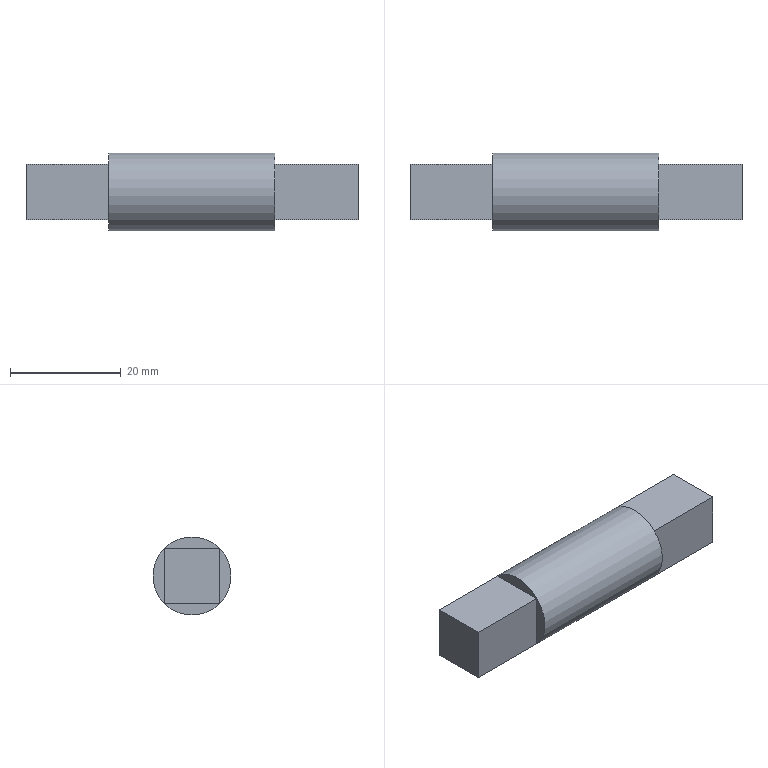Component | NX | 4 | 1 solid | 19 faces | box 60 x 14.14 x 14.14 mm | volume 7712 mm3 | plane 18 | cylinder 1 | commonest cylinder face diameters 14.142 x1
STEP:
#1=CARTESIAN_POINT('',(0.,0.,0.));
#2=DIRECTION('',(0.,0.,1.));
#3=DIRECTION('',(1.,0.,0.));
#4=AXIS2_PLACEMENT_3D('',#1,#2,#3);
#5=CARTESIAN_POINT('',(-30.,5.,43.));
#6=VERTEX_POINT('',#5);
#7=CARTESIAN_POINT('',(-15.,5.,43.));
#8=VERTEX_POINT('',#7);
#9=CARTESIAN_POINT('',(-30.,5.,43.));
#10=DIRECTION('',(1.,0.,0.));
#11=VECTOR('',#10,1.);
#12=LINE('',#9,#11);
#13=CARTESIAN_POINT('',(-30.,5.,43.));
#14=DIRECTION('',(0.,-1.,0.));
#15=DIRECTION('',(0.,0.,-1.));
#16=AXIS2_PLACEMENT_3D('',#13,#14,#15);
#17=PLANE('',#16);
#18=CARTESIAN_POINT('',(0.,0.));
#19=DIRECTION('',(0.,1.));
#20=VECTOR('',#19,1.);
#21=LINE('',#18,#20);
#22=(GEOMETRIC_REPRESENTATION_CONTEXT(2)PARAMETRIC_REPRESENTATION_CONTEXT()REPRESENTATION_CONTEXT('',''));
#23=DEFINITIONAL_REPRESENTATION('',(#21),#22);
#24=PCURVE('',#17,#23);
#25=CARTESIAN_POINT('',(-30.,-5.,43.));
#26=DIRECTION('',(0.,0.,-1.));
#27=DIRECTION('',(0.,1.,0.));
#28=AXIS2_PLACEMENT_3D('',#25,#26,#27);
#29=PLANE('',#28);
#30=CARTESIAN_POINT('',(10.,0.));
#31=DIRECTION('',(0.,1.));
#32=VECTOR('',#31,1.);
#33=LINE('',#30,#32);
#34=(GEOMETRIC_REPRESENTATION_CONTEXT(2)PARAMETRIC_REPRESENTATION_CONTEXT()REPRESENTATION_CONTEXT('',''));
#35=DEFINITIONAL_REPRESENTATION('',(#33),#34);
#36=PCURVE('',#29,#35);
#37=SURFACE_CURVE('',#12,(#24,#36),.PCURVE_S1.);
#38=EDGE_CURVE('',#6,#8,#37,.T.);
#39=ORIENTED_EDGE('',*,*,#38,.T.);
#40=CARTESIAN_POINT('',(-15.,5.,33.));
#41=VERTEX_POINT('',#40);
#42=CARTESIAN_POINT('',(-15.,5.,43.));
#43=DIRECTION('',(0.,0.,-1.));
#44=VECTOR('',#43,1.);
#45=LINE('',#42,#44);
#46=CARTESIAN_POINT('',(0.,15.));
#47=DIRECTION('',(1.,0.));
#48=VECTOR('',#47,1.);
#49=LINE('',#46,#48);
#50=(GEOMETRIC_REPRESENTATION_CONTEXT(2)PARAMETRIC_REPRESENTATION_CONTEXT()REPRESENTATION_CONTEXT('',''));
#51=DEFINITIONAL_REPRESENTATION('',(#49),#50);
#52=PCURVE('',#17,#51);
#53=CARTESIAN_POINT('',(-15.,0.,38.));
#54=DIRECTION('',(-1.,0.,0.));
#55=DIRECTION('',(0.,0.,-1.));
#56=AXIS2_PLACEMENT_3D('',#53,#54,#55);
#57=PLANE('',#56);
#58=CARTESIAN_POINT('',(-5.,-5.));
#59=DIRECTION('',(1.,0.));
#60=VECTOR('',#59,1.);
#61=LINE('',#58,#60);
#62=(GEOMETRIC_REPRESENTATION_CONTEXT(2)PARAMETRIC_REPRESENTATION_CONTEXT()REPRESENTATION_CONTEXT('',''));
#63=DEFINITIONAL_REPRESENTATION('',(#61),#62);
#64=PCURVE('',#57,#63);
#65=SURFACE_CURVE('',#45,(#52,#64),.PCURVE_S1.);
#66=EDGE_CURVE('',#8,#41,#65,.T.);
#67=ORIENTED_EDGE('',*,*,#66,.T.);
#68=CARTESIAN_POINT('',(-30.,5.,33.));
#69=VERTEX_POINT('',#68);
#70=CARTESIAN_POINT('',(-30.,5.,33.));
#71=DIRECTION('',(1.,0.,0.));
#72=VECTOR('',#71,1.);
#73=LINE('',#70,#72);
#74=CARTESIAN_POINT('',(10.,0.));
#75=DIRECTION('',(0.,1.));
#76=VECTOR('',#75,1.);
#77=LINE('',#74,#76);
#78=(GEOMETRIC_REPRESENTATION_CONTEXT(2)PARAMETRIC_REPRESENTATION_CONTEXT()REPRESENTATION_CONTEXT('',''));
#79=DEFINITIONAL_REPRESENTATION('',(#77),#78);
#80=PCURVE('',#17,#79);
#81=CARTESIAN_POINT('',(-30.,5.,33.));
#82=DIRECTION('',(0.,0.,1.));
#83=DIRECTION('',(0.,-1.,0.));
#84=AXIS2_PLACEMENT_3D('',#81,#82,#83);
#85=PLANE('',#84);
#86=CARTESIAN_POINT('',(0.,0.));
#87=DIRECTION('',(0.,1.));
#88=VECTOR('',#87,1.);
#89=LINE('',#86,#88);
#90=(GEOMETRIC_REPRESENTATION_CONTEXT(2)PARAMETRIC_REPRESENTATION_CONTEXT()REPRESENTATION_CONTEXT('',''));
#91=DEFINITIONAL_REPRESENTATION('',(#89),#90);
#92=PCURVE('',#85,#91);
#93=SURFACE_CURVE('',#73,(#80,#92),.PCURVE_S1.);
#94=EDGE_CURVE('',#69,#41,#93,.T.);
#95=ORIENTED_EDGE('',*,*,#94,.F.);
#96=CARTESIAN_POINT('',(-30.,5.,43.));
#97=DIRECTION('',(0.,0.,-1.));
#98=VECTOR('',#97,1.);
#99=LINE('',#96,#98);
#100=CARTESIAN_POINT('',(0.,0.));
#101=DIRECTION('',(1.,0.));
#102=VECTOR('',#101,1.);
#103=LINE('',#100,#102);
#104=(GEOMETRIC_REPRESENTATION_CONTEXT(2)PARAMETRIC_REPRESENTATION_CONTEXT()REPRESENTATION_CONTEXT('',''));
#105=DEFINITIONAL_REPRESENTATION('',(#103),#104);
#106=PCURVE('',#17,#105);
#107=CARTESIAN_POINT('',(-30.,0.,38.));
#108=DIRECTION('',(-1.,0.,0.));
#109=DIRECTION('',(0.,0.,-1.));
#110=AXIS2_PLACEMENT_3D('',#107,#108,#109);
#111=PLANE('',#110);
#112=CARTESIAN_POINT('',(-5.,-5.));
#113=DIRECTION('',(1.,0.));
#114=VECTOR('',#113,1.);
#115=LINE('',#112,#114);
#116=(GEOMETRIC_REPRESENTATION_CONTEXT(2)PARAMETRIC_REPRESENTATION_CONTEXT()REPRESENTATION_CONTEXT('',''));
#117=DEFINITIONAL_REPRESENTATION('',(#115),#116);
#118=PCURVE('',#111,#117);
#119=SURFACE_CURVE('',#99,(#106,#118),.PCURVE_S1.);
#120=EDGE_CURVE('',#6,#69,#119,.T.);
#121=ORIENTED_EDGE('',*,*,#120,.F.);
#122=EDGE_LOOP('',(#39,#67,#95,#121));
#123=FACE_BOUND('',#122,.T.);
#124=ADVANCED_FACE('',(#123),#17,.F.);
#125=ORIENTED_EDGE('',*,*,#94,.T.);
#126=CARTESIAN_POINT('',(-15.,-5.,33.));
#127=VERTEX_POINT('',#126);
#128=CARTESIAN_POINT('',(-15.,5.,33.));
#129=DIRECTION('',(0.,-1.,0.));
#130=VECTOR('',#129,1.);
#131=LINE('',#128,#130);
#132=CARTESIAN_POINT('',(0.,15.));
#133=DIRECTION('',(1.,0.));
#134=VECTOR('',#133,1.);
#135=LINE('',#132,#134);
#136=(GEOMETRIC_REPRESENTATION_CONTEXT(2)PARAMETRIC_REPRESENTATION_CONTEXT()REPRESENTATION_CONTEXT('',''));
#137=DEFINITIONAL_REPRESENTATION('',(#135),#136);
#138=PCURVE('',#85,#137);
#139=CARTESIAN_POINT('',(-15.,0.,38.));
#140=DIRECTION('',(-1.,0.,0.));
#141=DIRECTION('',(0.,0.,-1.));
#142=AXIS2_PLACEMENT_3D('',#139,#140,#141);
#143=PLANE('',#142);
#144=CARTESIAN_POINT('',(5.,-5.));
#145=DIRECTION('',(0.,1.));
#146=VECTOR('',#145,1.);
#147=LINE('',#144,#146);
#148=(GEOMETRIC_REPRESENTATION_CONTEXT(2)PARAMETRIC_REPRESENTATION_CONTEXT()REPRESENTATION_CONTEXT('',''));
#149=DEFINITIONAL_REPRESENTATION('',(#147),#148);
#150=PCURVE('',#143,#149);
#151=SURFACE_CURVE('',#131,(#138,#150),.PCURVE_S1.);
#152=EDGE_CURVE('',#41,#127,#151,.T.);
#153=ORIENTED_EDGE('',*,*,#152,.T.);
#154=CARTESIAN_POINT('',(-30.,-5.,33.));
#155=VERTEX_POINT('',#154);
#156=CARTESIAN_POINT('',(-30.,-5.,33.));
#157=DIRECTION('',(1.,0.,0.));
#158=VECTOR('',#157,1.);
#159=LINE('',#156,#158);
#160=CARTESIAN_POINT('',(10.,0.));
#161=DIRECTION('',(0.,1.));
#162=VECTOR('',#161,1.);
#163=LINE('',#160,#162);
#164=(GEOMETRIC_REPRESENTATION_CONTEXT(2)PARAMETRIC_REPRESENTATION_CONTEXT()REPRESENTATION_CONTEXT('',''));
#165=DEFINITIONAL_REPRESENTATION('',(#163),#164);
#166=PCURVE('',#85,#165);
#167=CARTESIAN_POINT('',(-30.,-5.,33.));
#168=DIRECTION('',(0.,1.,0.));
#169=DIRECTION('',(0.,0.,1.));
#170=AXIS2_PLACEMENT_3D('',#167,#168,#169);
#171=PLANE('',#170);
#172=CARTESIAN_POINT('',(0.,0.));
#173=DIRECTION('',(0.,1.));
#174=VECTOR('',#173,1.);
#175=LINE('',#172,#174);
#176=(GEOMETRIC_REPRESENTATION_CONTEXT(2)PARAMETRIC_REPRESENTATION_CONTEXT()REPRESENTATION_CONTEXT('',''));
#177=DEFINITIONAL_REPRESENTATION('',(#175),#176);
#178=PCURVE('',#171,#177);
#179=SURFACE_CURVE('',#159,(#166,#178),.PCURVE_S1.);
#180=EDGE_CURVE('',#155,#127,#179,.T.);
#181=ORIENTED_EDGE('',*,*,#180,.F.);
#182=CARTESIAN_POINT('',(-30.,5.,33.));
#183=DIRECTION('',(0.,-1.,0.));
#184=VECTOR('',#183,1.);
#185=LINE('',#182,#184);
#186=CARTESIAN_POINT('',(0.,0.));
#187=DIRECTION('',(1.,0.));
#188=VECTOR('',#187,1.);
#189=LINE('',#186,#188);
#190=(GEOMETRIC_REPRESENTATION_CONTEXT(2)PARAMETRIC_REPRESENTATION_CONTEXT()REPRESENTATION_CONTEXT('',''));
#191=DEFINITIONAL_REPRESENTATION('',(#189),#190);
#192=PCURVE('',#85,#191);
#193=CARTESIAN_POINT('',(5.,-5.));
#194=DIRECTION('',(0.,1.));
#195=VECTOR('',#194,1.);
#196=LINE('',#193,#195);
#197=(GEOMETRIC_REPRESENTATION_CONTEXT(2)PARAMETRIC_REPRESENTATION_CONTEXT()REPRESENTATION_CONTEXT('',''));
#198=DEFINITIONAL_REPRESENTATION('',(#196),#197);
#199=PCURVE('',#111,#198);
#200=SURFACE_CURVE('',#185,(#192,#199),.PCURVE_S1.);
#201=EDGE_CURVE('',#69,#155,#200,.T.);
#202=ORIENTED_EDGE('',*,*,#201,.F.);
#203=EDGE_LOOP('',(#125,#153,#181,#202));
#204=FACE_BOUND('',#203,.T.);
#205=ADVANCED_FACE('',(#204),#85,.F.);
#206=ORIENTED_EDGE('',*,*,#180,.T.);
#207=CARTESIAN_POINT('',(-15.,-5.,43.));
#208=VERTEX_POINT('',#207);
#209=CARTESIAN_POINT('',(-15.,-5.,33.));
#210=DIRECTION('',(0.,0.,1.));
#211=VECTOR('',#210,1.);
#212=LINE('',#209,#211);
#213=CARTESIAN_POINT('',(0.,15.));
#214=DIRECTION('',(1.,0.));
#215=VECTOR('',#214,1.);
#216=LINE('',#213,#215);
#217=(GEOMETRIC_REPRESENTATION_CONTEXT(2)PARAMETRIC_REPRESENTATION_CONTEXT()REPRESENTATION_CONTEXT('',''));
#218=DEFINITIONAL_REPRESENTATION('',(#216),#217);
#219=PCURVE('',#171,#218);
#220=CARTESIAN_POINT('',(-15.,0.,38.));
#221=DIRECTION('',(-1.,0.,0.));
#222=DIRECTION('',(0.,0.,-1.));
#223=AXIS2_PLACEMENT_3D('',#220,#221,#222);
#224=PLANE('',#223);
#225=CARTESIAN_POINT('',(5.,5.));
#226=DIRECTION('',(-1.,0.));
#227=VECTOR('',#226,1.);
#228=LINE('',#225,#227);
#229=(GEOMETRIC_REPRESENTATION_CONTEXT(2)PARAMETRIC_REPRESENTATION_CONTEXT()REPRESENTATION_CONTEXT('',''));
#230=DEFINITIONAL_REPRESENTATION('',(#228),#229);
#231=PCURVE('',#224,#230);
#232=SURFACE_CURVE('',#212,(#219,#231),.PCURVE_S1.);
#233=EDGE_CURVE('',#127,#208,#232,.T.);
#234=ORIENTED_EDGE('',*,*,#233,.T.);
#235=CARTESIAN_POINT('',(-30.,-5.,43.));
#236=VERTEX_POINT('',#235);
#237=CARTESIAN_POINT('',(-30.,-5.,43.));
#238=DIRECTION('',(1.,0.,0.));
#239=VECTOR('',#238,1.);
#240=LINE('',#237,#239);
#241=CARTESIAN_POINT('',(10.,0.));
#242=DIRECTION('',(0.,1.));
#243=VECTOR('',#242,1.);
#244=LINE('',#241,#243);
#245=(GEOMETRIC_REPRESENTATION_CONTEXT(2)PARAMETRIC_REPRESENTATION_CONTEXT()REPRESENTATION_CONTEXT('',''));
#246=DEFINITIONAL_REPRESENTATION('',(#244),#245);
#247=PCURVE('',#171,#246);
#248=CARTESIAN_POINT('',(0.,0.));
#249=DIRECTION('',(0.,1.));
#250=VECTOR('',#249,1.);
#251=LINE('',#248,#250);
#252=(GEOMETRIC_REPRESENTATION_CONTEXT(2)PARAMETRIC_REPRESENTATION_CONTEXT()REPRESENTATION_CONTEXT('',''));
#253=DEFINITIONAL_REPRESENTATION('',(#251),#252);
#254=PCURVE('',#29,#253);
#255=SURFACE_CURVE('',#240,(#247,#254),.PCURVE_S1.);
#256=EDGE_CURVE('',#236,#208,#255,.T.);
#257=ORIENTED_EDGE('',*,*,#256,.F.);
#258=CARTESIAN_POINT('',(-30.,-5.,33.));
#259=DIRECTION('',(0.,0.,1.));
#260=VECTOR('',#259,1.);
#261=LINE('',#258,#260);
#262=CARTESIAN_POINT('',(0.,0.));
#263=DIRECTION('',(1.,0.));
#264=VECTOR('',#263,1.);
#265=LINE('',#262,#264);
#266=(GEOMETRIC_REPRESENTATION_CONTEXT(2)PARAMETRIC_REPRESENTATION_CONTEXT()REPRESENTATION_CONTEXT('',''));
#267=DEFINITIONAL_REPRESENTATION('',(#265),#266);
#268=PCURVE('',#171,#267);
#269=CARTESIAN_POINT('',(5.,5.));
#270=DIRECTION('',(-1.,0.));
#271=VECTOR('',#270,1.);
#272=LINE('',#269,#271);
#273=(GEOMETRIC_REPRESENTATION_CONTEXT(2)PARAMETRIC_REPRESENTATION_CONTEXT()REPRESENTATION_CONTEXT('',''));
#274=DEFINITIONAL_REPRESENTATION('',(#272),#273);
#275=PCURVE('',#111,#274);
#276=SURFACE_CURVE('',#261,(#268,#275),.PCURVE_S1.);
#277=EDGE_CURVE('',#155,#236,#276,.T.);
#278=ORIENTED_EDGE('',*,*,#277,.F.);
#279=EDGE_LOOP('',(#206,#234,#257,#278));
#280=FACE_BOUND('',#279,.T.);
#281=ADVANCED_FACE('',(#280),#171,.F.);
#282=ORIENTED_EDGE('',*,*,#256,.T.);
#283=CARTESIAN_POINT('',(-15.,-5.,43.));
#284=DIRECTION('',(0.,1.,0.));
#285=VECTOR('',#284,1.);
#286=LINE('',#283,#285);
#287=CARTESIAN_POINT('',(0.,15.));
#288=DIRECTION('',(1.,0.));
#289=VECTOR('',#288,1.);
#290=LINE('',#287,#289);
#291=(GEOMETRIC_REPRESENTATION_CONTEXT(2)PARAMETRIC_REPRESENTATION_CONTEXT()REPRESENTATION_CONTEXT('',''));
#292=DEFINITIONAL_REPRESENTATION('',(#290),#291);
#293=PCURVE('',#29,#292);
#294=CARTESIAN_POINT('',(-15.,0.,38.));
#295=DIRECTION('',(-1.,0.,0.));
#296=DIRECTION('',(0.,0.,-1.));
#297=AXIS2_PLACEMENT_3D('',#294,#295,#296);
#298=PLANE('',#297);
#299=CARTESIAN_POINT('',(-5.,5.));
#300=DIRECTION('',(0.,-1.));
#301=VECTOR('',#300,1.);
#302=LINE('',#299,#301);
#303=(GEOMETRIC_REPRESENTATION_CONTEXT(2)PARAMETRIC_REPRESENTATION_CONTEXT()REPRESENTATION_CONTEXT('',''));
#304=DEFINITIONAL_REPRESENTATION('',(#302),#303);
#305=PCURVE('',#298,#304);
#306=SURFACE_CURVE('',#286,(#293,#305),.PCURVE_S1.);
#307=EDGE_CURVE('',#208,#8,#306,.T.);
#308=ORIENTED_EDGE('',*,*,#307,.T.);
#309=ORIENTED_EDGE('',*,*,#38,.F.);
#310=CARTESIAN_POINT('',(-30.,-5.,43.));
#311=DIRECTION('',(0.,1.,0.));
#312=VECTOR('',#311,1.);
#313=LINE('',#310,#312);
#314=CARTESIAN_POINT('',(0.,0.));
#315=DIRECTION('',(1.,0.));
#316=VECTOR('',#315,1.);
#317=LINE('',#314,#316);
#318=(GEOMETRIC_REPRESENTATION_CONTEXT(2)PARAMETRIC_REPRESENTATION_CONTEXT()REPRESENTATION_CONTEXT('',''));
#319=DEFINITIONAL_REPRESENTATION('',(#317),#318);
#320=PCURVE('',#29,#319);
#321=CARTESIAN_POINT('',(-5.,5.));
#322=DIRECTION('',(0.,-1.));
#323=VECTOR('',#322,1.);
#324=LINE('',#321,#323);
#325=(GEOMETRIC_REPRESENTATION_CONTEXT(2)PARAMETRIC_REPRESENTATION_CONTEXT()REPRESENTATION_CONTEXT('',''));
#326=DEFINITIONAL_REPRESENTATION('',(#324),#325);
#327=PCURVE('',#111,#326);
#328=SURFACE_CURVE('',#313,(#320,#327),.PCURVE_S1.);
#329=EDGE_CURVE('',#236,#6,#328,.T.);
#330=ORIENTED_EDGE('',*,*,#329,.F.);
#331=EDGE_LOOP('',(#282,#308,#309,#330));
#332=FACE_BOUND('',#331,.T.);
#333=ADVANCED_FACE('',(#332),#29,.F.);
#334=ORIENTED_EDGE('',*,*,#120,.T.);
#335=ORIENTED_EDGE('',*,*,#201,.T.);
#336=ORIENTED_EDGE('',*,*,#277,.T.);
#337=ORIENTED_EDGE('',*,*,#329,.T.);
#338=EDGE_LOOP('',(#334,#335,#336,#337));
#339=FACE_BOUND('',#338,.T.);
#340=ADVANCED_FACE('',(#339),#111,.T.);
#341=ORIENTED_EDGE('',*,*,#66,.F.);
#342=CARTESIAN_POINT('',(-15.,0.,38.));
#343=DIRECTION('',(1.,0.,0.));
#344=DIRECTION('',(0.,0.,-1.));
#345=AXIS2_PLACEMENT_3D('',#342,#343,#344);
#346=CIRCLE('',#345,7.071);
#347=CARTESIAN_POINT('',(7.071,0.));
#348=CARTESIAN_POINT('',(7.071,-12.247));
#349=CARTESIAN_POINT('',(-3.536,-6.124));
#350=CARTESIAN_POINT('',(-14.142,-0.));
#351=CARTESIAN_POINT('',(-3.536,6.124));
#352=CARTESIAN_POINT('',(7.071,12.247));
#353=CARTESIAN_POINT('',(7.071,0.));
#354=(BOUNDED_CURVE()B_SPLINE_CURVE(2,(#347,#348,#349,#350,#351,#352,#353),.UNSPECIFIED.,.T.,.F.)B_SPLINE_CURVE_WITH_KNOTS((1,2,2,2,2,1),(-2.094,0.,2.094,4.189,6.283,8.378),.UNSPECIFIED.)CURVE()GEOMETRIC_REPRESENTATION_ITEM()RATIONAL_B_SPLINE_CURVE((1.,0.5,1.,0.5,1.,0.5,1.))REPRESENTATION_ITEM(''));
#355=(GEOMETRIC_REPRESENTATION_CONTEXT(2)PARAMETRIC_REPRESENTATION_CONTEXT()REPRESENTATION_CONTEXT('',''));
#356=DEFINITIONAL_REPRESENTATION('',(#354),#355);
#357=PCURVE('',#57,#356);
#358=CARTESIAN_POINT('',(30.,0.,38.));
#359=DIRECTION('',(-1.,0.,0.));
#360=DIRECTION('',(0.,0.,1.));
#361=AXIS2_PLACEMENT_3D('',#358,#359,#360);
#362=CYLINDRICAL_SURFACE('',#361,7.071);
#363=CARTESIAN_POINT('',(3.142,45.));
#364=DIRECTION('',(-1.,0.));
#365=VECTOR('',#364,1.);
#366=LINE('',#363,#365);
#367=(GEOMETRIC_REPRESENTATION_CONTEXT(2)PARAMETRIC_REPRESENTATION_CONTEXT()REPRESENTATION_CONTEXT('',''));
#368=DEFINITIONAL_REPRESENTATION('',(#366),#367);
#369=PCURVE('',#362,#368);
#370=SURFACE_CURVE('',#346,(#357,#369),.PCURVE_S1.);
#371=EDGE_CURVE('',#41,#8,#370,.T.);
#372=ORIENTED_EDGE('',*,*,#371,.F.);
#373=EDGE_LOOP('',(#341,#372));
#374=FACE_BOUND('',#373,.T.);
#375=ADVANCED_FACE('',(#374),#57,.T.);
#376=ORIENTED_EDGE('',*,*,#152,.F.);
#377=CARTESIAN_POINT('',(-15.,0.,38.));
#378=DIRECTION('',(1.,0.,0.));
#379=DIRECTION('',(0.,0.,-1.));
#380=AXIS2_PLACEMENT_3D('',#377,#378,#379);
#381=CIRCLE('',#380,7.071);
#382=CARTESIAN_POINT('',(7.071,0.));
#383=CARTESIAN_POINT('',(7.071,-12.247));
#384=CARTESIAN_POINT('',(-3.536,-6.124));
#385=CARTESIAN_POINT('',(-14.142,-0.));
#386=CARTESIAN_POINT('',(-3.536,6.124));
#387=CARTESIAN_POINT('',(7.071,12.247));
#388=CARTESIAN_POINT('',(7.071,0.));
#389=(BOUNDED_CURVE()B_SPLINE_CURVE(2,(#382,#383,#384,#385,#386,#387,#388),.UNSPECIFIED.,.T.,.F.)B_SPLINE_CURVE_WITH_KNOTS((1,2,2,2,2,1),(-2.094,0.,2.094,4.189,6.283,8.378),.UNSPECIFIED.)CURVE()GEOMETRIC_REPRESENTATION_ITEM()RATIONAL_B_SPLINE_CURVE((1.,0.5,1.,0.5,1.,0.5,1.))REPRESENTATION_ITEM(''));
#390=(GEOMETRIC_REPRESENTATION_CONTEXT(2)PARAMETRIC_REPRESENTATION_CONTEXT()REPRESENTATION_CONTEXT('',''));
#391=DEFINITIONAL_REPRESENTATION('',(#389),#390);
#392=PCURVE('',#143,#391);
#393=CARTESIAN_POINT('',(9.425,45.));
#394=DIRECTION('',(-1.,0.));
#395=VECTOR('',#394,1.);
#396=LINE('',#393,#395);
#397=(GEOMETRIC_REPRESENTATION_CONTEXT(2)PARAMETRIC_REPRESENTATION_CONTEXT()REPRESENTATION_CONTEXT('',''));
#398=DEFINITIONAL_REPRESENTATION('',(#396),#397);
#399=PCURVE('',#362,#398);
#400=SURFACE_CURVE('',#381,(#392,#399),.PCURVE_S1.);
#401=EDGE_CURVE('',#127,#41,#400,.T.);
#402=ORIENTED_EDGE('',*,*,#401,.F.);
#403=EDGE_LOOP('',(#376,#402));
#404=FACE_BOUND('',#403,.T.);
#405=ADVANCED_FACE('',(#404),#143,.T.);
#406=ORIENTED_EDGE('',*,*,#233,.F.);
#407=CARTESIAN_POINT('',(-15.,0.,38.));
#408=DIRECTION('',(1.,0.,0.));
#409=DIRECTION('',(0.,0.,-1.));
#410=AXIS2_PLACEMENT_3D('',#407,#408,#409);
#411=CIRCLE('',#410,7.071);
#412=CARTESIAN_POINT('',(7.071,0.));
#413=CARTESIAN_POINT('',(7.071,-12.247));
#414=CARTESIAN_POINT('',(-3.536,-6.124));
#415=CARTESIAN_POINT('',(-14.142,-0.));
#416=CARTESIAN_POINT('',(-3.536,6.124));
#417=CARTESIAN_POINT('',(7.071,12.247));
#418=CARTESIAN_POINT('',(7.071,0.));
#419=(BOUNDED_CURVE()B_SPLINE_CURVE(2,(#412,#413,#414,#415,#416,#417,#418),.UNSPECIFIED.,.T.,.F.)B_SPLINE_CURVE_WITH_KNOTS((1,2,2,2,2,1),(-2.094,0.,2.094,4.189,6.283,8.378),.UNSPECIFIED.)CURVE()GEOMETRIC_REPRESENTATION_ITEM()RATIONAL_B_SPLINE_CURVE((1.,0.5,1.,0.5,1.,0.5,1.))REPRESENTATION_ITEM(''));
#420=(GEOMETRIC_REPRESENTATION_CONTEXT(2)PARAMETRIC_REPRESENTATION_CONTEXT()REPRESENTATION_CONTEXT('',''));
#421=DEFINITIONAL_REPRESENTATION('',(#419),#420);
#422=PCURVE('',#224,#421);
#423=CARTESIAN_POINT('',(9.425,45.));
#424=DIRECTION('',(-1.,0.));
#425=VECTOR('',#424,1.);
#426=LINE('',#423,#425);
#427=(GEOMETRIC_REPRESENTATION_CONTEXT(2)PARAMETRIC_REPRESENTATION_CONTEXT()REPRESENTATION_CONTEXT('',''));
#428=DEFINITIONAL_REPRESENTATION('',(#426),#427);
#429=PCURVE('',#362,#428);
#430=SURFACE_CURVE('',#411,(#422,#429),.PCURVE_S1.);
#431=EDGE_CURVE('',#208,#127,#430,.T.);
#432=ORIENTED_EDGE('',*,*,#431,.F.);
#433=EDGE_LOOP('',(#406,#432));
#434=FACE_BOUND('',#433,.T.);
#435=ADVANCED_FACE('',(#434),#224,.T.);
#436=ORIENTED_EDGE('',*,*,#307,.F.);
#437=CARTESIAN_POINT('',(-15.,0.,38.));
#438=DIRECTION('',(1.,0.,0.));
#439=DIRECTION('',(0.,0.,-1.));
#440=AXIS2_PLACEMENT_3D('',#437,#438,#439);
#441=CIRCLE('',#440,7.071);
#442=CARTESIAN_POINT('',(7.071,0.));
#443=CARTESIAN_POINT('',(7.071,-12.247));
#444=CARTESIAN_POINT('',(-3.536,-6.124));
#445=CARTESIAN_POINT('',(-14.142,-0.));
#446=CARTESIAN_POINT('',(-3.536,6.124));
#447=CARTESIAN_POINT('',(7.071,12.247));
#448=CARTESIAN_POINT('',(7.071,0.));
#449=(BOUNDED_CURVE()B_SPLINE_CURVE(2,(#442,#443,#444,#445,#446,#447,#448),.UNSPECIFIED.,.T.,.F.)B_SPLINE_CURVE_WITH_KNOTS((1,2,2,2,2,1),(-2.094,0.,2.094,4.189,6.283,8.378),.UNSPECIFIED.)CURVE()GEOMETRIC_REPRESENTATION_ITEM()RATIONAL_B_SPLINE_CURVE((1.,0.5,1.,0.5,1.,0.5,1.))REPRESENTATION_ITEM(''));
#450=(GEOMETRIC_REPRESENTATION_CONTEXT(2)PARAMETRIC_REPRESENTATION_CONTEXT()REPRESENTATION_CONTEXT('',''));
#451=DEFINITIONAL_REPRESENTATION('',(#449),#450);
#452=PCURVE('',#298,#451);
#453=CARTESIAN_POINT('',(9.425,45.));
#454=DIRECTION('',(-1.,0.));
#455=VECTOR('',#454,1.);
#456=LINE('',#453,#455);
#457=(GEOMETRIC_REPRESENTATION_CONTEXT(2)PARAMETRIC_REPRESENTATION_CONTEXT()REPRESENTATION_CONTEXT('',''));
#458=DEFINITIONAL_REPRESENTATION('',(#456),#457);
#459=PCURVE('',#362,#458);
#460=SURFACE_CURVE('',#441,(#452,#459),.PCURVE_S1.);
#461=EDGE_CURVE('',#8,#208,#460,.T.);
#462=ORIENTED_EDGE('',*,*,#461,.F.);
#463=EDGE_LOOP('',(#436,#462));
#464=FACE_BOUND('',#463,.T.);
#465=ADVANCED_FACE('',(#464),#298,.T.);
#466=CARTESIAN_POINT('',(15.,5.,33.));
#467=VERTEX_POINT('',#466);
#468=CARTESIAN_POINT('',(15.,5.,43.));
#469=VERTEX_POINT('',#468);
#470=CARTESIAN_POINT('',(15.,5.,43.));
#471=DIRECTION('',(0.,0.,1.));
#472=VECTOR('',#471,1.);
#473=LINE('',#470,#472);
#474=CARTESIAN_POINT('',(15.,0.,38.));
#475=DIRECTION('',(1.,0.,0.));
#476=DIRECTION('',(0.,0.,1.));
#477=AXIS2_PLACEMENT_3D('',#474,#475,#476);
#478=PLANE('',#477);
#479=CARTESIAN_POINT('',(5.,-5.));
#480=DIRECTION('',(1.,0.));
#481=VECTOR('',#480,1.);
#482=LINE('',#479,#481);
#483=(GEOMETRIC_REPRESENTATION_CONTEXT(2)PARAMETRIC_REPRESENTATION_CONTEXT()REPRESENTATION_CONTEXT('',''));
#484=DEFINITIONAL_REPRESENTATION('',(#482),#483);
#485=PCURVE('',#478,#484);
#486=CARTESIAN_POINT('',(-30.,5.,43.));
#487=DIRECTION('',(0.,-1.,0.));
#488=DIRECTION('',(0.,0.,-1.));
#489=AXIS2_PLACEMENT_3D('',#486,#487,#488);
#490=PLANE('',#489);
#491=CARTESIAN_POINT('',(0.,45.));
#492=DIRECTION('',(-1.,0.));
#493=VECTOR('',#492,1.);
#494=LINE('',#491,#493);
#495=(GEOMETRIC_REPRESENTATION_CONTEXT(2)PARAMETRIC_REPRESENTATION_CONTEXT()REPRESENTATION_CONTEXT('',''));
#496=DEFINITIONAL_REPRESENTATION('',(#494),#495);
#497=PCURVE('',#490,#496);
#498=SURFACE_CURVE('',#473,(#485,#497),.PCURVE_S1.);
#499=EDGE_CURVE('',#467,#469,#498,.T.);
#500=ORIENTED_EDGE('',*,*,#499,.F.);
#501=CARTESIAN_POINT('',(15.,0.,38.));
#502=DIRECTION('',(-1.,0.,0.));
#503=DIRECTION('',(0.,0.,1.));
#504=AXIS2_PLACEMENT_3D('',#501,#502,#503);
#505=CIRCLE('',#504,7.071);
#506=CARTESIAN_POINT('',(7.071,0.));
#507=CARTESIAN_POINT('',(7.071,-12.247));
#508=CARTESIAN_POINT('',(-3.536,-6.124));
#509=CARTESIAN_POINT('',(-14.142,-0.));
#510=CARTESIAN_POINT('',(-3.536,6.124));
#511=CARTESIAN_POINT('',(7.071,12.247));
#512=CARTESIAN_POINT('',(7.071,0.));
#513=(BOUNDED_CURVE()B_SPLINE_CURVE(2,(#506,#507,#508,#509,#510,#511,#512),.UNSPECIFIED.,.T.,.F.)B_SPLINE_CURVE_WITH_KNOTS((1,2,2,2,2,1),(-2.094,0.,2.094,4.189,6.283,8.378),.UNSPECIFIED.)CURVE()GEOMETRIC_REPRESENTATION_ITEM()RATIONAL_B_SPLINE_CURVE((1.,0.5,1.,0.5,1.,0.5,1.))REPRESENTATION_ITEM(''));
#514=(GEOMETRIC_REPRESENTATION_CONTEXT(2)PARAMETRIC_REPRESENTATION_CONTEXT()REPRESENTATION_CONTEXT('',''));
#515=DEFINITIONAL_REPRESENTATION('',(#513),#514);
#516=PCURVE('',#478,#515);
#517=CARTESIAN_POINT('',(0.,15.));
#518=DIRECTION('',(1.,0.));
#519=VECTOR('',#518,1.);
#520=LINE('',#517,#519);
#521=(GEOMETRIC_REPRESENTATION_CONTEXT(2)PARAMETRIC_REPRESENTATION_CONTEXT()REPRESENTATION_CONTEXT('',''));
#522=DEFINITIONAL_REPRESENTATION('',(#520),#521);
#523=PCURVE('',#362,#522);
#524=SURFACE_CURVE('',#505,(#516,#523),.PCURVE_S1.);
#525=EDGE_CURVE('',#469,#467,#524,.T.);
#526=ORIENTED_EDGE('',*,*,#525,.F.);
#527=EDGE_LOOP('',(#500,#526));
#528=FACE_BOUND('',#527,.T.);
#529=ADVANCED_FACE('',(#528),#478,.T.);
#530=CARTESIAN_POINT('',(15.,-5.,33.));
#531=VERTEX_POINT('',#530);
#532=CARTESIAN_POINT('',(15.,5.,33.));
#533=DIRECTION('',(0.,1.,0.));
#534=VECTOR('',#533,1.);
#535=LINE('',#532,#534);
#536=CARTESIAN_POINT('',(15.,0.,38.));
#537=DIRECTION('',(1.,0.,0.));
#538=DIRECTION('',(0.,0.,1.));
#539=AXIS2_PLACEMENT_3D('',#536,#537,#538);
#540=PLANE('',#539);
#541=CARTESIAN_POINT('',(-5.,-5.));
#542=DIRECTION('',(0.,-1.));
#543=VECTOR('',#542,1.);
#544=LINE('',#541,#543);
#545=(GEOMETRIC_REPRESENTATION_CONTEXT(2)PARAMETRIC_REPRESENTATION_CONTEXT()REPRESENTATION_CONTEXT('',''));
#546=DEFINITIONAL_REPRESENTATION('',(#544),#545);
#547=PCURVE('',#540,#546);
#548=CARTESIAN_POINT('',(-30.,5.,33.));
#549=DIRECTION('',(0.,0.,1.));
#550=DIRECTION('',(0.,-1.,0.));
#551=AXIS2_PLACEMENT_3D('',#548,#549,#550);
#552=PLANE('',#551);
#553=CARTESIAN_POINT('',(0.,45.));
#554=DIRECTION('',(-1.,0.));
#555=VECTOR('',#554,1.);
#556=LINE('',#553,#555);
#557=(GEOMETRIC_REPRESENTATION_CONTEXT(2)PARAMETRIC_REPRESENTATION_CONTEXT()REPRESENTATION_CONTEXT('',''));
#558=DEFINITIONAL_REPRESENTATION('',(#556),#557);
#559=PCURVE('',#552,#558);
#560=SURFACE_CURVE('',#535,(#547,#559),.PCURVE_S1.);
#561=EDGE_CURVE('',#531,#467,#560,.T.);
#562=ORIENTED_EDGE('',*,*,#561,.F.);
#563=CARTESIAN_POINT('',(15.,0.,38.));
#564=DIRECTION('',(-1.,0.,0.));
#565=DIRECTION('',(0.,0.,1.));
#566=AXIS2_PLACEMENT_3D('',#563,#564,#565);
#567=CIRCLE('',#566,7.071);
#568=CARTESIAN_POINT('',(7.071,0.));
#569=CARTESIAN_POINT('',(7.071,-12.247));
#570=CARTESIAN_POINT('',(-3.536,-6.124));
#571=CARTESIAN_POINT('',(-14.142,-0.));
#572=CARTESIAN_POINT('',(-3.536,6.124));
#573=CARTESIAN_POINT('',(7.071,12.247));
#574=CARTESIAN_POINT('',(7.071,0.));
#575=(BOUNDED_CURVE()B_SPLINE_CURVE(2,(#568,#569,#570,#571,#572,#573,#574),.UNSPECIFIED.,.T.,.F.)B_SPLINE_CURVE_WITH_KNOTS((1,2,2,2,2,1),(-2.094,0.,2.094,4.189,6.283,8.378),.UNSPECIFIED.)CURVE()GEOMETRIC_REPRESENTATION_ITEM()RATIONAL_B_SPLINE_CURVE((1.,0.5,1.,0.5,1.,0.5,1.))REPRESENTATION_ITEM(''));
#576=(GEOMETRIC_REPRESENTATION_CONTEXT(2)PARAMETRIC_REPRESENTATION_CONTEXT()REPRESENTATION_CONTEXT('',''));
#577=DEFINITIONAL_REPRESENTATION('',(#575),#576);
#578=PCURVE('',#540,#577);
#579=CARTESIAN_POINT('',(0.,15.));
#580=DIRECTION('',(1.,0.));
#581=VECTOR('',#580,1.);
#582=LINE('',#579,#581);
#583=(GEOMETRIC_REPRESENTATION_CONTEXT(2)PARAMETRIC_REPRESENTATION_CONTEXT()REPRESENTATION_CONTEXT('',''));
#584=DEFINITIONAL_REPRESENTATION('',(#582),#583);
#585=PCURVE('',#362,#584);
#586=SURFACE_CURVE('',#567,(#578,#585),.PCURVE_S1.);
#587=EDGE_CURVE('',#467,#531,#586,.T.);
#588=ORIENTED_EDGE('',*,*,#587,.F.);
#589=EDGE_LOOP('',(#562,#588));
#590=FACE_BOUND('',#589,.T.);
#591=ADVANCED_FACE('',(#590),#540,.T.);
#592=CARTESIAN_POINT('',(15.,-5.,43.));
#593=VERTEX_POINT('',#592);
#594=CARTESIAN_POINT('',(15.,-5.,33.));
#595=DIRECTION('',(0.,0.,-1.));
#596=VECTOR('',#595,1.);
#597=LINE('',#594,#596);
#598=CARTESIAN_POINT('',(15.,0.,38.));
#599=DIRECTION('',(1.,0.,0.));
#600=DIRECTION('',(0.,0.,1.));
#601=AXIS2_PLACEMENT_3D('',#598,#599,#600);
#602=PLANE('',#601);
#603=CARTESIAN_POINT('',(-5.,5.));
#604=DIRECTION('',(-1.,0.));
#605=VECTOR('',#604,1.);
#606=LINE('',#603,#605);
#607=(GEOMETRIC_REPRESENTATION_CONTEXT(2)PARAMETRIC_REPRESENTATION_CONTEXT()REPRESENTATION_CONTEXT('',''));
#608=DEFINITIONAL_REPRESENTATION('',(#606),#607);
#609=PCURVE('',#602,#608);
#610=CARTESIAN_POINT('',(-30.,-5.,33.));
#611=DIRECTION('',(0.,1.,0.));
#612=DIRECTION('',(0.,0.,1.));
#613=AXIS2_PLACEMENT_3D('',#610,#611,#612);
#614=PLANE('',#613);
#615=CARTESIAN_POINT('',(0.,45.));
#616=DIRECTION('',(-1.,0.));
#617=VECTOR('',#616,1.);
#618=LINE('',#615,#617);
#619=(GEOMETRIC_REPRESENTATION_CONTEXT(2)PARAMETRIC_REPRESENTATION_CONTEXT()REPRESENTATION_CONTEXT('',''));
#620=DEFINITIONAL_REPRESENTATION('',(#618),#619);
#621=PCURVE('',#614,#620);
#622=SURFACE_CURVE('',#597,(#609,#621),.PCURVE_S1.);
#623=EDGE_CURVE('',#593,#531,#622,.T.);
#624=ORIENTED_EDGE('',*,*,#623,.F.);
#625=CARTESIAN_POINT('',(15.,0.,38.));
#626=DIRECTION('',(-1.,0.,0.));
#627=DIRECTION('',(0.,0.,1.));
#628=AXIS2_PLACEMENT_3D('',#625,#626,#627);
#629=CIRCLE('',#628,7.071);
#630=CARTESIAN_POINT('',(7.071,0.));
#631=CARTESIAN_POINT('',(7.071,-12.247));
#632=CARTESIAN_POINT('',(-3.536,-6.124));
#633=CARTESIAN_POINT('',(-14.142,-0.));
#634=CARTESIAN_POINT('',(-3.536,6.124));
#635=CARTESIAN_POINT('',(7.071,12.247));
#636=CARTESIAN_POINT('',(7.071,0.));
#637=(BOUNDED_CURVE()B_SPLINE_CURVE(2,(#630,#631,#632,#633,#634,#635,#636),.UNSPECIFIED.,.T.,.F.)B_SPLINE_CURVE_WITH_KNOTS((1,2,2,2,2,1),(-2.094,0.,2.094,4.189,6.283,8.378),.UNSPECIFIED.)CURVE()GEOMETRIC_REPRESENTATION_ITEM()RATIONAL_B_SPLINE_CURVE((1.,0.5,1.,0.5,1.,0.5,1.))REPRESENTATION_ITEM(''));
#638=(GEOMETRIC_REPRESENTATION_CONTEXT(2)PARAMETRIC_REPRESENTATION_CONTEXT()REPRESENTATION_CONTEXT('',''));
#639=DEFINITIONAL_REPRESENTATION('',(#637),#638);
#640=PCURVE('',#602,#639);
#641=CARTESIAN_POINT('',(0.,15.));
#642=DIRECTION('',(1.,0.));
#643=VECTOR('',#642,1.);
#644=LINE('',#641,#643);
#645=(GEOMETRIC_REPRESENTATION_CONTEXT(2)PARAMETRIC_REPRESENTATION_CONTEXT()REPRESENTATION_CONTEXT('',''));
#646=DEFINITIONAL_REPRESENTATION('',(#644),#645);
#647=PCURVE('',#362,#646);
#648=SURFACE_CURVE('',#629,(#640,#647),.PCURVE_S1.);
#649=EDGE_CURVE('',#531,#593,#648,.T.);
#650=ORIENTED_EDGE('',*,*,#649,.F.);
#651=EDGE_LOOP('',(#624,#650));
#652=FACE_BOUND('',#651,.T.);
#653=ADVANCED_FACE('',(#652),#602,.T.);
#654=CARTESIAN_POINT('',(15.,-5.,43.));
#655=DIRECTION('',(0.,-1.,0.));
#656=VECTOR('',#655,1.);
#657=LINE('',#654,#656);
#658=CARTESIAN_POINT('',(15.,0.,38.));
#659=DIRECTION('',(1.,0.,0.));
#660=DIRECTION('',(0.,0.,1.));
#661=AXIS2_PLACEMENT_3D('',#658,#659,#660);
#662=PLANE('',#661);
#663=CARTESIAN_POINT('',(5.,5.));
#664=DIRECTION('',(0.,1.));
#665=VECTOR('',#664,1.);
#666=LINE('',#663,#665);
#667=(GEOMETRIC_REPRESENTATION_CONTEXT(2)PARAMETRIC_REPRESENTATION_CONTEXT()REPRESENTATION_CONTEXT('',''));
#668=DEFINITIONAL_REPRESENTATION('',(#666),#667);
#669=PCURVE('',#662,#668);
#670=CARTESIAN_POINT('',(-30.,-5.,43.));
#671=DIRECTION('',(0.,0.,-1.));
#672=DIRECTION('',(0.,1.,0.));
#673=AXIS2_PLACEMENT_3D('',#670,#671,#672);
#674=PLANE('',#673);
#675=CARTESIAN_POINT('',(0.,45.));
#676=DIRECTION('',(-1.,0.));
#677=VECTOR('',#676,1.);
#678=LINE('',#675,#677);
#679=(GEOMETRIC_REPRESENTATION_CONTEXT(2)PARAMETRIC_REPRESENTATION_CONTEXT()REPRESENTATION_CONTEXT('',''));
#680=DEFINITIONAL_REPRESENTATION('',(#678),#679);
#681=PCURVE('',#674,#680);
#682=SURFACE_CURVE('',#657,(#669,#681),.PCURVE_S1.);
#683=EDGE_CURVE('',#469,#593,#682,.T.);
#684=ORIENTED_EDGE('',*,*,#683,.F.);
#685=CARTESIAN_POINT('',(15.,0.,38.));
#686=DIRECTION('',(-1.,0.,0.));
#687=DIRECTION('',(0.,0.,1.));
#688=AXIS2_PLACEMENT_3D('',#685,#686,#687);
#689=CIRCLE('',#688,7.071);
#690=CARTESIAN_POINT('',(7.071,0.));
#691=CARTESIAN_POINT('',(7.071,-12.247));
#692=CARTESIAN_POINT('',(-3.536,-6.124));
#693=CARTESIAN_POINT('',(-14.142,-0.));
#694=CARTESIAN_POINT('',(-3.536,6.124));
#695=CARTESIAN_POINT('',(7.071,12.247));
#696=CARTESIAN_POINT('',(7.071,0.));
#697=(BOUNDED_CURVE()B_SPLINE_CURVE(2,(#690,#691,#692,#693,#694,#695,#696),.UNSPECIFIED.,.T.,.F.)B_SPLINE_CURVE_WITH_KNOTS((1,2,2,2,2,1),(-2.094,0.,2.094,4.189,6.283,8.378),.UNSPECIFIED.)CURVE()GEOMETRIC_REPRESENTATION_ITEM()RATIONAL_B_SPLINE_CURVE((1.,0.5,1.,0.5,1.,0.5,1.))REPRESENTATION_ITEM(''));
#698=(GEOMETRIC_REPRESENTATION_CONTEXT(2)PARAMETRIC_REPRESENTATION_CONTEXT()REPRESENTATION_CONTEXT('',''));
#699=DEFINITIONAL_REPRESENTATION('',(#697),#698);
#700=PCURVE('',#662,#699);
#701=CARTESIAN_POINT('',(-0.,15.));
#702=DIRECTION('',(1.,0.));
#703=VECTOR('',#702,1.);
#704=LINE('',#701,#703);
#705=(GEOMETRIC_REPRESENTATION_CONTEXT(2)PARAMETRIC_REPRESENTATION_CONTEXT()REPRESENTATION_CONTEXT('',''));
#706=DEFINITIONAL_REPRESENTATION('',(#704),#705);
#707=PCURVE('',#362,#706);
#708=SURFACE_CURVE('',#689,(#700,#707),.PCURVE_S1.);
#709=EDGE_CURVE('',#593,#469,#708,.T.);
#710=ORIENTED_EDGE('',*,*,#709,.F.);
#711=EDGE_LOOP('',(#684,#710));
#712=FACE_BOUND('',#711,.T.);
#713=ADVANCED_FACE('',(#712),#662,.T.);
#714=ORIENTED_EDGE('',*,*,#401,.T.);
#715=ORIENTED_EDGE('',*,*,#371,.T.);
#716=CARTESIAN_POINT('',(15.,5.,43.));
#717=CARTESIAN_POINT('',(-15.,5.,43.));
#718=B_SPLINE_CURVE_WITH_KNOTS('',1,(#716,#717),.UNSPECIFIED.,.F.,.F.,(2,2),(15.,45.),.PIECEWISE_BEZIER_KNOTS.);
#719=CARTESIAN_POINT('',(0.7854,0.));
#720=DIRECTION('',(0.,1.));
#721=VECTOR('',#720,1.);
#722=LINE('',#719,#721);
#723=(GEOMETRIC_REPRESENTATION_CONTEXT(2)PARAMETRIC_REPRESENTATION_CONTEXT()REPRESENTATION_CONTEXT('',''));
#724=DEFINITIONAL_REPRESENTATION('',(#722),#723);
#725=PCURVE('',#362,#724);
#726=CARTESIAN_POINT('',(7.069,0.));
#727=DIRECTION('',(0.,1.));
#728=VECTOR('',#727,1.);
#729=LINE('',#726,#728);
#730=(GEOMETRIC_REPRESENTATION_CONTEXT(2)PARAMETRIC_REPRESENTATION_CONTEXT()REPRESENTATION_CONTEXT('',''));
#731=DEFINITIONAL_REPRESENTATION('',(#729),#730);
#732=PCURVE('',#362,#731);
#733=SEAM_CURVE('',#718,(#725,#732),.PCURVE_S1.);
#734=EDGE_CURVE('',#469,#8,#733,.T.);
#735=ORIENTED_EDGE('',*,*,#734,.F.);
#736=ORIENTED_EDGE('',*,*,#525,.T.);
#737=ORIENTED_EDGE('',*,*,#587,.T.);
#738=ORIENTED_EDGE('',*,*,#649,.T.);
#739=ORIENTED_EDGE('',*,*,#709,.T.);
#740=ORIENTED_EDGE('',*,*,#734,.T.);
#741=ORIENTED_EDGE('',*,*,#461,.T.);
#742=ORIENTED_EDGE('',*,*,#431,.T.);
#743=EDGE_LOOP('',(#714,#715,#735,#736,#737,#738,#739,#740,#741,#742));
#744=FACE_BOUND('',#743,.T.);
#745=ADVANCED_FACE('',(#744),#362,.T.);
#746=CARTESIAN_POINT('',(30.,5.,43.));
#747=VERTEX_POINT('',#746);
#748=CARTESIAN_POINT('',(30.,5.,33.));
#749=VERTEX_POINT('',#748);
#750=CARTESIAN_POINT('',(30.,5.,43.));
#751=DIRECTION('',(0.,0.,-1.));
#752=VECTOR('',#751,1.);
#753=LINE('',#750,#752);
#754=CARTESIAN_POINT('',(30.,0.,38.));
#755=DIRECTION('',(-1.,0.,0.));
#756=DIRECTION('',(0.,0.,-1.));
#757=AXIS2_PLACEMENT_3D('',#754,#755,#756);
#758=PLANE('',#757);
#759=CARTESIAN_POINT('',(-5.,-5.));
#760=DIRECTION('',(1.,0.));
#761=VECTOR('',#760,1.);
#762=LINE('',#759,#761);
#763=(GEOMETRIC_REPRESENTATION_CONTEXT(2)PARAMETRIC_REPRESENTATION_CONTEXT()REPRESENTATION_CONTEXT('',''));
#764=DEFINITIONAL_REPRESENTATION('',(#762),#763);
#765=PCURVE('',#758,#764);
#766=CARTESIAN_POINT('',(0.,60.));
#767=DIRECTION('',(1.,0.));
#768=VECTOR('',#767,1.);
#769=LINE('',#766,#768);
#770=(GEOMETRIC_REPRESENTATION_CONTEXT(2)PARAMETRIC_REPRESENTATION_CONTEXT()REPRESENTATION_CONTEXT('',''));
#771=DEFINITIONAL_REPRESENTATION('',(#769),#770);
#772=PCURVE('',#490,#771);
#773=SURFACE_CURVE('',#753,(#765,#772),.PCURVE_S1.);
#774=EDGE_CURVE('',#747,#749,#773,.T.);
#775=ORIENTED_EDGE('',*,*,#774,.F.);
#776=CARTESIAN_POINT('',(30.,-5.,43.));
#777=VERTEX_POINT('',#776);
#778=CARTESIAN_POINT('',(30.,-5.,43.));
#779=DIRECTION('',(0.,1.,0.));
#780=VECTOR('',#779,1.);
#781=LINE('',#778,#780);
#782=CARTESIAN_POINT('',(-5.,5.));
#783=DIRECTION('',(0.,-1.));
#784=VECTOR('',#783,1.);
#785=LINE('',#782,#784);
#786=(GEOMETRIC_REPRESENTATION_CONTEXT(2)PARAMETRIC_REPRESENTATION_CONTEXT()REPRESENTATION_CONTEXT('',''));
#787=DEFINITIONAL_REPRESENTATION('',(#785),#786);
#788=PCURVE('',#758,#787);
#789=CARTESIAN_POINT('',(0.,60.));
#790=DIRECTION('',(1.,0.));
#791=VECTOR('',#790,1.);
#792=LINE('',#789,#791);
#793=(GEOMETRIC_REPRESENTATION_CONTEXT(2)PARAMETRIC_REPRESENTATION_CONTEXT()REPRESENTATION_CONTEXT('',''));
#794=DEFINITIONAL_REPRESENTATION('',(#792),#793);
#795=PCURVE('',#674,#794);
#796=SURFACE_CURVE('',#781,(#788,#795),.PCURVE_S1.);
#797=EDGE_CURVE('',#777,#747,#796,.T.);
#798=ORIENTED_EDGE('',*,*,#797,.F.);
#799=CARTESIAN_POINT('',(30.,-5.,33.));
#800=VERTEX_POINT('',#799);
#801=CARTESIAN_POINT('',(30.,-5.,33.));
#802=DIRECTION('',(0.,0.,1.));
#803=VECTOR('',#802,1.);
#804=LINE('',#801,#803);
#805=CARTESIAN_POINT('',(5.,5.));
#806=DIRECTION('',(-1.,0.));
#807=VECTOR('',#806,1.);
#808=LINE('',#805,#807);
#809=(GEOMETRIC_REPRESENTATION_CONTEXT(2)PARAMETRIC_REPRESENTATION_CONTEXT()REPRESENTATION_CONTEXT('',''));
#810=DEFINITIONAL_REPRESENTATION('',(#808),#809);
#811=PCURVE('',#758,#810);
#812=CARTESIAN_POINT('',(0.,60.));
#813=DIRECTION('',(1.,0.));
#814=VECTOR('',#813,1.);
#815=LINE('',#812,#814);
#816=(GEOMETRIC_REPRESENTATION_CONTEXT(2)PARAMETRIC_REPRESENTATION_CONTEXT()REPRESENTATION_CONTEXT('',''));
#817=DEFINITIONAL_REPRESENTATION('',(#815),#816);
#818=PCURVE('',#614,#817);
#819=SURFACE_CURVE('',#804,(#811,#818),.PCURVE_S1.);
#820=EDGE_CURVE('',#800,#777,#819,.T.);
#821=ORIENTED_EDGE('',*,*,#820,.F.);
#822=CARTESIAN_POINT('',(30.,5.,33.));
#823=DIRECTION('',(0.,-1.,0.));
#824=VECTOR('',#823,1.);
#825=LINE('',#822,#824);
#826=CARTESIAN_POINT('',(5.,-5.));
#827=DIRECTION('',(0.,1.));
#828=VECTOR('',#827,1.);
#829=LINE('',#826,#828);
#830=(GEOMETRIC_REPRESENTATION_CONTEXT(2)PARAMETRIC_REPRESENTATION_CONTEXT()REPRESENTATION_CONTEXT('',''));
#831=DEFINITIONAL_REPRESENTATION('',(#829),#830);
#832=PCURVE('',#758,#831);
#833=CARTESIAN_POINT('',(0.,60.));
#834=DIRECTION('',(1.,0.));
#835=VECTOR('',#834,1.);
#836=LINE('',#833,#835);
#837=(GEOMETRIC_REPRESENTATION_CONTEXT(2)PARAMETRIC_REPRESENTATION_CONTEXT()REPRESENTATION_CONTEXT('',''));
#838=DEFINITIONAL_REPRESENTATION('',(#836),#837);
#839=PCURVE('',#552,#838);
#840=SURFACE_CURVE('',#825,(#832,#839),.PCURVE_S1.);
#841=EDGE_CURVE('',#749,#800,#840,.T.);
#842=ORIENTED_EDGE('',*,*,#841,.F.);
#843=EDGE_LOOP('',(#775,#798,#821,#842));
#844=FACE_BOUND('',#843,.T.);
#845=ADVANCED_FACE('',(#844),#758,.F.);
#846=CARTESIAN_POINT('',(-30.,5.,43.));
#847=DIRECTION('',(1.,0.,0.));
#848=VECTOR('',#847,1.);
#849=LINE('',#846,#848);
#850=CARTESIAN_POINT('',(10.,0.));
#851=DIRECTION('',(0.,1.));
#852=VECTOR('',#851,1.);
#853=LINE('',#850,#852);
#854=(GEOMETRIC_REPRESENTATION_CONTEXT(2)PARAMETRIC_REPRESENTATION_CONTEXT()REPRESENTATION_CONTEXT('',''));
#855=DEFINITIONAL_REPRESENTATION('',(#853),#854);
#856=PCURVE('',#674,#855);
#857=CARTESIAN_POINT('',(0.,0.));
#858=DIRECTION('',(0.,1.));
#859=VECTOR('',#858,1.);
#860=LINE('',#857,#859);
#861=(GEOMETRIC_REPRESENTATION_CONTEXT(2)PARAMETRIC_REPRESENTATION_CONTEXT()REPRESENTATION_CONTEXT('',''));
#862=DEFINITIONAL_REPRESENTATION('',(#860),#861);
#863=PCURVE('',#490,#862);
#864=SURFACE_CURVE('',#849,(#856,#863),.PCURVE_S1.);
#865=EDGE_CURVE('',#469,#747,#864,.T.);
#866=ORIENTED_EDGE('',*,*,#865,.F.);
#867=ORIENTED_EDGE('',*,*,#683,.T.);
#868=CARTESIAN_POINT('',(-30.,-5.,43.));
#869=DIRECTION('',(1.,0.,0.));
#870=VECTOR('',#869,1.);
#871=LINE('',#868,#870);
#872=CARTESIAN_POINT('',(0.,0.));
#873=DIRECTION('',(0.,1.));
#874=VECTOR('',#873,1.);
#875=LINE('',#872,#874);
#876=(GEOMETRIC_REPRESENTATION_CONTEXT(2)PARAMETRIC_REPRESENTATION_CONTEXT()REPRESENTATION_CONTEXT('',''));
#877=DEFINITIONAL_REPRESENTATION('',(#875),#876);
#878=PCURVE('',#674,#877);
#879=CARTESIAN_POINT('',(10.,0.));
#880=DIRECTION('',(0.,1.));
#881=VECTOR('',#880,1.);
#882=LINE('',#879,#881);
#883=(GEOMETRIC_REPRESENTATION_CONTEXT(2)PARAMETRIC_REPRESENTATION_CONTEXT()REPRESENTATION_CONTEXT('',''));
#884=DEFINITIONAL_REPRESENTATION('',(#882),#883);
#885=PCURVE('',#614,#884);
#886=SURFACE_CURVE('',#871,(#878,#885),.PCURVE_S1.);
#887=EDGE_CURVE('',#593,#777,#886,.T.);
#888=ORIENTED_EDGE('',*,*,#887,.T.);
#889=ORIENTED_EDGE('',*,*,#797,.T.);
#890=EDGE_LOOP('',(#866,#867,#888,#889));
#891=FACE_BOUND('',#890,.T.);
#892=ADVANCED_FACE('',(#891),#674,.F.);
#893=ORIENTED_EDGE('',*,*,#887,.F.);
#894=ORIENTED_EDGE('',*,*,#623,.T.);
#895=CARTESIAN_POINT('',(-30.,-5.,33.));
#896=DIRECTION('',(1.,0.,0.));
#897=VECTOR('',#896,1.);
#898=LINE('',#895,#897);
#899=CARTESIAN_POINT('',(0.,0.));
#900=DIRECTION('',(0.,1.));
#901=VECTOR('',#900,1.);
#902=LINE('',#899,#901);
#903=(GEOMETRIC_REPRESENTATION_CONTEXT(2)PARAMETRIC_REPRESENTATION_CONTEXT()REPRESENTATION_CONTEXT('',''));
#904=DEFINITIONAL_REPRESENTATION('',(#902),#903);
#905=PCURVE('',#614,#904);
#906=CARTESIAN_POINT('',(10.,0.));
#907=DIRECTION('',(0.,1.));
#908=VECTOR('',#907,1.);
#909=LINE('',#906,#908);
#910=(GEOMETRIC_REPRESENTATION_CONTEXT(2)PARAMETRIC_REPRESENTATION_CONTEXT()REPRESENTATION_CONTEXT('',''));
#911=DEFINITIONAL_REPRESENTATION('',(#909),#910);
#912=PCURVE('',#552,#911);
#913=SURFACE_CURVE('',#898,(#905,#912),.PCURVE_S1.);
#914=EDGE_CURVE('',#531,#800,#913,.T.);
#915=ORIENTED_EDGE('',*,*,#914,.T.);
#916=ORIENTED_EDGE('',*,*,#820,.T.);
#917=EDGE_LOOP('',(#893,#894,#915,#916));
#918=FACE_BOUND('',#917,.T.);
#919=ADVANCED_FACE('',(#918),#614,.F.);
#920=ORIENTED_EDGE('',*,*,#914,.F.);
#921=ORIENTED_EDGE('',*,*,#561,.T.);
#922=CARTESIAN_POINT('',(-30.,5.,33.));
#923=DIRECTION('',(1.,0.,0.));
#924=VECTOR('',#923,1.);
#925=LINE('',#922,#924);
#926=CARTESIAN_POINT('',(0.,0.));
#927=DIRECTION('',(0.,1.));
#928=VECTOR('',#927,1.);
#929=LINE('',#926,#928);
#930=(GEOMETRIC_REPRESENTATION_CONTEXT(2)PARAMETRIC_REPRESENTATION_CONTEXT()REPRESENTATION_CONTEXT('',''));
#931=DEFINITIONAL_REPRESENTATION('',(#929),#930);
#932=PCURVE('',#552,#931);
#933=CARTESIAN_POINT('',(10.,0.));
#934=DIRECTION('',(0.,1.));
#935=VECTOR('',#934,1.);
#936=LINE('',#933,#935);
#937=(GEOMETRIC_REPRESENTATION_CONTEXT(2)PARAMETRIC_REPRESENTATION_CONTEXT()REPRESENTATION_CONTEXT('',''));
#938=DEFINITIONAL_REPRESENTATION('',(#936),#937);
#939=PCURVE('',#490,#938);
#940=SURFACE_CURVE('',#925,(#932,#939),.PCURVE_S1.);
#941=EDGE_CURVE('',#467,#749,#940,.T.);
#942=ORIENTED_EDGE('',*,*,#941,.T.);
#943=ORIENTED_EDGE('',*,*,#841,.T.);
#944=EDGE_LOOP('',(#920,#921,#942,#943));
#945=FACE_BOUND('',#944,.T.);
#946=ADVANCED_FACE('',(#945),#552,.F.);
#947=ORIENTED_EDGE('',*,*,#941,.F.);
#948=ORIENTED_EDGE('',*,*,#499,.T.);
#949=ORIENTED_EDGE('',*,*,#865,.T.);
#950=ORIENTED_EDGE('',*,*,#774,.T.);
#951=EDGE_LOOP('',(#947,#948,#949,#950));
#952=FACE_BOUND('',#951,.T.);
#953=ADVANCED_FACE('',(#952),#490,.F.);
#954=CLOSED_SHELL('',(#124,#205,#281,#333,#340,#375,#405,#435,#465,#529,#591,#653,#713,#745,#845,#892,#919,#946,#953));
#955=MANIFOLD_SOLID_BREP('',#954);
#956=(LENGTH_UNIT()NAMED_UNIT(*)SI_UNIT(.MILLI.,.METRE.));
#957=UNCERTAINTY_MEASURE_WITH_UNIT(LENGTH_MEASURE(0.000001),#956,'','');
#958=(NAMED_UNIT(*)PLANE_ANGLE_UNIT()SI_UNIT($,.RADIAN.));
#959=(NAMED_UNIT(*)SI_UNIT($,.STERADIAN.)SOLID_ANGLE_UNIT());
#960=(GEOMETRIC_REPRESENTATION_CONTEXT(3)GLOBAL_UNCERTAINTY_ASSIGNED_CONTEXT((#957))GLOBAL_UNIT_ASSIGNED_CONTEXT((#956,#958,#959))REPRESENTATION_CONTEXT('',''));
#961=ADVANCED_BREP_SHAPE_REPRESENTATION('',(#4,#955),#960);